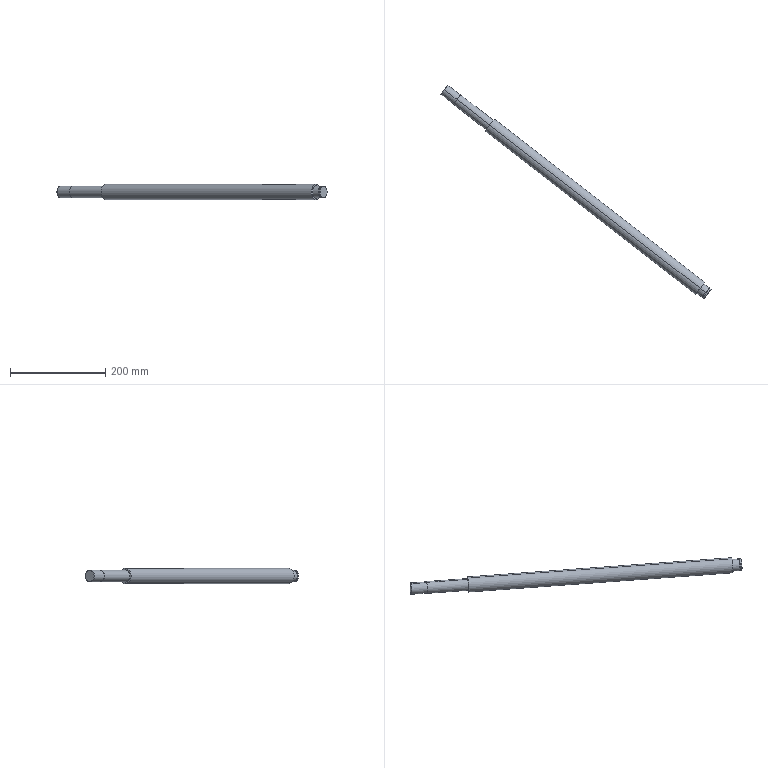Component | SolidWorks | MISUMI_BSSRK3210-800-F34-P20-1_SHAFT_MISUMI_BSSRK3210-800-F34-P20-1 | 1 solid | 27 faces | box 567.36 x 447.98 x 32 mm | volume 517409 mm3 | cylinder 12 | plane 7 | cone 4 | torus 4 | commonest cylinder face diameters 25 x6 24 x2 23.9 x2 32 x2
build123d program:
from build123d import *

# Parameters (mm, degrees)
FILLET1_R     = 0.3
FILLET2_R     = 0.5
CHAMFER1_SIZE = 0.5


with BuildPart() as part:
    # Sketch1 → Revolve1 (revolve)
    with BuildSketch(Plane.XY, mode=Mode.PRIVATE) as revolve1_sk:
        Polygon((0, 0), (700, 0), (700, 12), (666, 12), (666, 12.5), (579, 12.5), (579, 16), (20, 16), (20, 12.5), (5, 12.5), (5, 11.95), (3.65, 11.95), (3.65, 12.5), (0, 12.5), align=None)
    revolve(revolve1_sk.sketch.rotate(Axis((0, 0, 0), (1, 0, 0)), 90), axis=Axis((0, 0, 0), (1, 0, 0)))

    # Fillet1
    fillet1_edges = [part.edges().sort_by_distance(p)[0] for p in [
        (579, 0, -12.5),
    ]]
    fillet(fillet1_edges, radius=FILLET1_R)

    # Fillet2
    fillet2_edges = [part.edges().sort_by_distance(p)[0] for p in [
        (20, 0, -12.5),
    ]]
    fillet(fillet2_edges, radius=FILLET2_R)

    # Chamfer1
    chamfer1_edges = [part.edges().sort_by_distance(p)[0] for p in [
        (700, 0, -12),
        (0, 0, -12.5),
    ]]
    chamfer(chamfer1_edges, length=CHAMFER1_SIZE)


solid = part.part

# Placed as in the assembly
solid = solid.moved(Location((382.255, 447.91, 276.411), (0.7035, -0.5461, 142.183)))
STEP:
#1=COLOUR_RGB('',0.7922,0.8196,0.9333);
#2=FILL_AREA_STYLE_COLOUR('',#1);
#3=FILL_AREA_STYLE('',(#2));
#4=SURFACE_STYLE_FILL_AREA(#3);
#5=SURFACE_SIDE_STYLE('',(#4));
#6=SURFACE_STYLE_USAGE(.BOTH.,#5);
#7=PRESENTATION_STYLE_ASSIGNMENT((#6));
#8=CARTESIAN_POINT('',(15.049,17.634,11.355));
#9=VERTEX_POINT('',#8);
#10=CARTESIAN_POINT('',(15.049,17.634,10.41));
#11=VERTEX_POINT('',#10);
#12=CARTESIAN_POINT('',(15.049,17.634,10.882));
#13=DIRECTION('',(0.7899,-0.6132,-0.));
#14=DIRECTION('',(0.,0.,-1.));
#15=AXIS2_PLACEMENT_3D('',#12,#13,#14);
#16=CIRCLE('',#15,0.4724);
#17=EDGE_CURVE('',#9,#11,#16,.T.);
#18=ORIENTED_EDGE('',*,*,#17,.F.);
#19=CARTESIAN_POINT('',(15.034,17.646,11.374));
#20=VERTEX_POINT('',#19);
#21=CARTESIAN_POINT('',(15.049,17.634,11.355));
#22=DIRECTION('',(-0.5586,0.4336,0.7071));
#23=VECTOR('',#22,39.37);
#24=LINE('',#21,#23);
#25=EDGE_CURVE('',#9,#20,#24,.T.);
#26=ORIENTED_EDGE('',*,*,#25,.T.);
#27=CARTESIAN_POINT('',(15.034,17.646,10.39));
#28=VERTEX_POINT('',#27);
#29=CARTESIAN_POINT('',(15.034,17.646,10.882));
#30=DIRECTION('',(-0.7899,0.6132,0.));
#31=DIRECTION('',(0.,0.,-1.));
#32=AXIS2_PLACEMENT_3D('',#29,#30,#31);
#33=CIRCLE('',#32,0.4921);
#34=EDGE_CURVE('',#28,#20,#33,.T.);
#35=ORIENTED_EDGE('',*,*,#34,.F.);
#36=CARTESIAN_POINT('',(15.049,17.634,10.41));
#37=DIRECTION('',(-0.5586,0.4336,-0.7071));
#38=VECTOR('',#37,39.37);
#39=LINE('',#36,#38);
#40=EDGE_CURVE('',#11,#28,#39,.T.);
#41=ORIENTED_EDGE('',*,*,#40,.F.);
#42=EDGE_LOOP('',(#18,#26,#35,#41));
#43=FACE_OUTER_BOUND('',#42,.T.);
#44=CARTESIAN_POINT('',(15.049,17.634,10.882));
#45=DIRECTION('',(-0.7899,0.6132,0.));
#46=DIRECTION('',(0.,0.,-1.));
#47=AXIS2_PLACEMENT_3D('',#44,#45,#46);
#48=CONICAL_SURFACE('',#47,0.4724,0.7854);
#49=ADVANCED_FACE('',(#43),#48,.T.);
#50=CARTESIAN_POINT('',(-6.72,34.533,10.43));
#51=VERTEX_POINT('',#50);
#52=CARTESIAN_POINT('',(-6.72,34.533,11.335));
#53=VERTEX_POINT('',#52);
#54=CARTESIAN_POINT('',(-6.72,34.533,10.882));
#55=DIRECTION('',(-0.7899,0.6132,0.));
#56=DIRECTION('',(-0.,-0.,1.));
#57=AXIS2_PLACEMENT_3D('',#54,#55,#56);
#58=CIRCLE('',#57,0.4528);
#59=EDGE_CURVE('',#51,#53,#58,.T.);
#60=ORIENTED_EDGE('',*,*,#59,.F.);
#61=CARTESIAN_POINT('',(-6.705,34.521,10.41));
#62=VERTEX_POINT('',#61);
#63=CARTESIAN_POINT('',(-6.705,34.521,10.41));
#64=DIRECTION('',(0.5586,-0.4336,-0.7071));
#65=VECTOR('',#64,39.37);
#66=LINE('',#63,#65);
#67=EDGE_CURVE('',#51,#62,#66,.T.);
#68=ORIENTED_EDGE('',*,*,#67,.T.);
#69=CARTESIAN_POINT('',(-6.705,34.521,11.355));
#70=VERTEX_POINT('',#69);
#71=CARTESIAN_POINT('',(-6.705,34.521,10.882));
#72=DIRECTION('',(0.7899,-0.6132,-0.));
#73=DIRECTION('',(-0.,-0.,1.));
#74=AXIS2_PLACEMENT_3D('',#71,#72,#73);
#75=CIRCLE('',#74,0.4724);
#76=EDGE_CURVE('',#70,#62,#75,.T.);
#77=ORIENTED_EDGE('',*,*,#76,.F.);
#78=CARTESIAN_POINT('',(-6.705,34.521,11.355));
#79=DIRECTION('',(0.5586,-0.4336,0.7071));
#80=VECTOR('',#79,39.37);
#81=LINE('',#78,#80);
#82=EDGE_CURVE('',#53,#70,#81,.T.);
#83=ORIENTED_EDGE('',*,*,#82,.F.);
#84=EDGE_LOOP('',(#60,#68,#77,#83));
#85=FACE_OUTER_BOUND('',#84,.T.);
#86=CARTESIAN_POINT('',(-6.705,34.521,10.882));
#87=DIRECTION('',(0.7899,-0.6132,-0.));
#88=DIRECTION('',(-0.,-0.,1.));
#89=AXIS2_PLACEMENT_3D('',#86,#87,#88);
#90=CONICAL_SURFACE('',#89,0.4724,0.7854);
#91=ADVANCED_FACE('',(#85),#90,.T.);
#92=CARTESIAN_POINT('',(14.427,18.117,11.394));
#93=VERTEX_POINT('',#92);
#94=CARTESIAN_POINT('',(14.427,18.117,10.371));
#95=VERTEX_POINT('',#94);
#96=CARTESIAN_POINT('',(14.427,18.117,10.882));
#97=DIRECTION('',(-0.7899,0.6132,0.));
#98=DIRECTION('',(0.,0.,-1.));
#99=AXIS2_PLACEMENT_3D('',#96,#97,#98);
#100=CIRCLE('',#99,0.5118);
#101=EDGE_CURVE('',#93,#95,#100,.T.);
#102=ORIENTED_EDGE('',*,*,#101,.F.);
#103=CARTESIAN_POINT('',(14.443,18.105,11.374));
#104=VERTEX_POINT('',#103);
#105=CARTESIAN_POINT('',(14.443,18.105,11.394));
#106=DIRECTION('',(-0.6132,-0.7899,-0.));
#107=DIRECTION('',(0.7899,-0.6132,0.));
#108=AXIS2_PLACEMENT_3D('',#105,#106,#107);
#109=CIRCLE('',#108,0.01969);
#110=EDGE_CURVE('',#93,#104,#109,.T.);
#111=ORIENTED_EDGE('',*,*,#110,.T.);
#112=CARTESIAN_POINT('',(14.443,18.105,10.39));
#113=VERTEX_POINT('',#112);
#114=CARTESIAN_POINT('',(14.443,18.105,10.882));
#115=DIRECTION('',(0.7899,-0.6132,-0.));
#116=DIRECTION('',(0.,0.,-1.));
#117=AXIS2_PLACEMENT_3D('',#114,#115,#116);
#118=CIRCLE('',#117,0.4921);
#119=EDGE_CURVE('',#113,#104,#118,.T.);
#120=ORIENTED_EDGE('',*,*,#119,.F.);
#121=CARTESIAN_POINT('',(14.443,18.105,10.371));
#122=DIRECTION('',(0.6132,0.7899,0.));
#123=DIRECTION('',(-0.7899,0.6132,0.));
#124=AXIS2_PLACEMENT_3D('',#121,#122,#123);
#125=CIRCLE('',#124,0.01969);
#126=EDGE_CURVE('',#95,#113,#125,.T.);
#127=ORIENTED_EDGE('',*,*,#126,.F.);
#128=EDGE_LOOP('',(#102,#111,#120,#127));
#129=FACE_OUTER_BOUND('',#128,.T.);
#130=CARTESIAN_POINT('',(14.443,18.105,10.882));
#131=DIRECTION('',(-0.7899,0.6132,0.));
#132=DIRECTION('',(0.,0.,-1.));
#133=AXIS2_PLACEMENT_3D('',#130,#131,#132);
#134=TOROIDAL_SURFACE('',#133,0.5118,0.01969);
#135=ADVANCED_FACE('',(#129),#134,.F.);
#136=CARTESIAN_POINT('',(-2.957,31.612,10.378));
#137=VERTEX_POINT('',#136);
#138=CARTESIAN_POINT('',(-2.957,31.612,11.386));
#139=VERTEX_POINT('',#138);
#140=CARTESIAN_POINT('',(-2.957,31.612,10.882));
#141=DIRECTION('',(0.7899,-0.6132,-0.));
#142=DIRECTION('',(-0.,-0.,1.));
#143=AXIS2_PLACEMENT_3D('',#140,#141,#142);
#144=CIRCLE('',#143,0.5039);
#145=EDGE_CURVE('',#137,#139,#144,.T.);
#146=ORIENTED_EDGE('',*,*,#145,.F.);
#147=CARTESIAN_POINT('',(-2.967,31.619,10.39));
#148=VERTEX_POINT('',#147);
#149=CARTESIAN_POINT('',(-2.967,31.619,10.378));
#150=DIRECTION('',(-0.6132,-0.7899,-0.));
#151=DIRECTION('',(0.7899,-0.6132,0.));
#152=AXIS2_PLACEMENT_3D('',#149,#150,#151);
#153=CIRCLE('',#152,0.01181);
#154=EDGE_CURVE('',#137,#148,#153,.T.);
#155=ORIENTED_EDGE('',*,*,#154,.T.);
#156=CARTESIAN_POINT('',(-2.967,31.619,11.374));
#157=VERTEX_POINT('',#156);
#158=CARTESIAN_POINT('',(-2.967,31.619,10.882));
#159=DIRECTION('',(-0.7899,0.6132,0.));
#160=DIRECTION('',(-0.,-0.,1.));
#161=AXIS2_PLACEMENT_3D('',#158,#159,#160);
#162=CIRCLE('',#161,0.4921);
#163=EDGE_CURVE('',#157,#148,#162,.T.);
#164=ORIENTED_EDGE('',*,*,#163,.F.);
#165=CARTESIAN_POINT('',(-2.967,31.619,11.386));
#166=DIRECTION('',(0.6132,0.7899,0.));
#167=DIRECTION('',(-0.7899,0.6132,0.));
#168=AXIS2_PLACEMENT_3D('',#165,#166,#167);
#169=CIRCLE('',#168,0.01181);
#170=EDGE_CURVE('',#139,#157,#169,.T.);
#171=ORIENTED_EDGE('',*,*,#170,.F.);
#172=EDGE_LOOP('',(#146,#155,#164,#171));
#173=FACE_OUTER_BOUND('',#172,.T.);
#174=CARTESIAN_POINT('',(-2.967,31.619,10.882));
#175=DIRECTION('',(0.7899,-0.6132,-0.));
#176=DIRECTION('',(-0.,-0.,1.));
#177=AXIS2_PLACEMENT_3D('',#174,#175,#176);
#178=TOROIDAL_SURFACE('',#177,0.5039,0.01181);
#179=ADVANCED_FACE('',(#173),#178,.F.);
#180=CARTESIAN_POINT('',(-5.663,33.713,11.374));
#181=VERTEX_POINT('',#180);
#182=CARTESIAN_POINT('',(-5.663,33.713,10.39));
#183=VERTEX_POINT('',#182);
#184=CARTESIAN_POINT('',(-5.663,33.713,10.882));
#185=DIRECTION('',(0.7899,-0.6132,-0.));
#186=DIRECTION('',(-0.,-0.,1.));
#187=AXIS2_PLACEMENT_3D('',#184,#185,#186);
#188=CIRCLE('',#187,0.4921);
#189=EDGE_CURVE('',#181,#183,#188,.T.);
#190=ORIENTED_EDGE('',*,*,#189,.T.);
#191=CARTESIAN_POINT('',(15.049,17.634,10.39));
#192=DIRECTION('',(0.7899,-0.6132,-0.));
#193=VECTOR('',#192,39.37);
#194=LINE('',#191,#193);
#195=EDGE_CURVE('',#183,#148,#194,.T.);
#196=ORIENTED_EDGE('',*,*,#195,.T.);
#197=CARTESIAN_POINT('',(-2.967,31.619,10.882));
#198=DIRECTION('',(-0.7899,0.6132,0.));
#199=DIRECTION('',(-0.,-0.,1.));
#200=AXIS2_PLACEMENT_3D('',#197,#198,#199);
#201=CIRCLE('',#200,0.4921);
#202=EDGE_CURVE('',#148,#157,#201,.T.);
#203=ORIENTED_EDGE('',*,*,#202,.T.);
#204=CARTESIAN_POINT('',(15.049,17.634,11.374));
#205=DIRECTION('',(0.7899,-0.6132,-0.));
#206=VECTOR('',#205,39.37);
#207=LINE('',#204,#206);
#208=EDGE_CURVE('',#181,#157,#207,.T.);
#209=ORIENTED_EDGE('',*,*,#208,.F.);
#210=EDGE_LOOP('',(#190,#196,#203,#209));
#211=FACE_OUTER_BOUND('',#210,.T.);
#212=CARTESIAN_POINT('',(15.049,17.634,10.882));
#213=DIRECTION('',(0.7899,-0.6132,-0.));
#214=DIRECTION('',(-0.,-0.,1.));
#215=AXIS2_PLACEMENT_3D('',#212,#213,#214);
#216=CYLINDRICAL_SURFACE('',#215,0.4921);
#217=ADVANCED_FACE('',(#211),#216,.T.);
#218=ORIENTED_EDGE('',*,*,#76,.T.);
#219=CARTESIAN_POINT('',(-5.663,33.713,10.41));
#220=VERTEX_POINT('',#219);
#221=CARTESIAN_POINT('',(15.049,17.634,10.41));
#222=DIRECTION('',(0.7899,-0.6132,-0.));
#223=VECTOR('',#222,39.37);
#224=LINE('',#221,#223);
#225=EDGE_CURVE('',#62,#220,#224,.T.);
#226=ORIENTED_EDGE('',*,*,#225,.T.);
#227=CARTESIAN_POINT('',(-5.663,33.713,11.355));
#228=VERTEX_POINT('',#227);
#229=CARTESIAN_POINT('',(-5.663,33.713,10.882));
#230=DIRECTION('',(0.7899,-0.6132,-0.));
#231=DIRECTION('',(-0.,-0.,1.));
#232=AXIS2_PLACEMENT_3D('',#229,#230,#231);
#233=CIRCLE('',#232,0.4724);
#234=EDGE_CURVE('',#228,#220,#233,.T.);
#235=ORIENTED_EDGE('',*,*,#234,.F.);
#236=CARTESIAN_POINT('',(15.049,17.634,11.355));
#237=DIRECTION('',(0.7899,-0.6132,-0.));
#238=VECTOR('',#237,39.37);
#239=LINE('',#236,#238);
#240=EDGE_CURVE('',#70,#228,#239,.T.);
#241=ORIENTED_EDGE('',*,*,#240,.F.);
#242=EDGE_LOOP('',(#218,#226,#235,#241));
#243=FACE_OUTER_BOUND('',#242,.T.);
#244=CARTESIAN_POINT('',(15.049,17.634,10.882));
#245=DIRECTION('',(0.7899,-0.6132,-0.));
#246=DIRECTION('',(-0.,-0.,1.));
#247=AXIS2_PLACEMENT_3D('',#244,#245,#246);
#248=CYLINDRICAL_SURFACE('',#247,0.4724);
#249=ADVANCED_FACE('',(#243),#248,.T.);
#250=CARTESIAN_POINT('',(14.936,17.722,11.374));
#251=VERTEX_POINT('',#250);
#252=CARTESIAN_POINT('',(14.936,17.722,10.39));
#253=VERTEX_POINT('',#252);
#254=CARTESIAN_POINT('',(14.936,17.722,10.882));
#255=DIRECTION('',(0.7899,-0.6132,-0.));
#256=DIRECTION('',(-0.,-0.,1.));
#257=AXIS2_PLACEMENT_3D('',#254,#255,#256);
#258=CIRCLE('',#257,0.4921);
#259=EDGE_CURVE('',#251,#253,#258,.T.);
#260=ORIENTED_EDGE('',*,*,#259,.T.);
#261=CARTESIAN_POINT('',(15.049,17.634,10.39));
#262=DIRECTION('',(0.7899,-0.6132,-0.));
#263=VECTOR('',#262,39.37);
#264=LINE('',#261,#263);
#265=EDGE_CURVE('',#253,#28,#264,.T.);
#266=ORIENTED_EDGE('',*,*,#265,.T.);
#267=ORIENTED_EDGE('',*,*,#34,.T.);
#268=CARTESIAN_POINT('',(15.049,17.634,11.374));
#269=DIRECTION('',(0.7899,-0.6132,-0.));
#270=VECTOR('',#269,39.37);
#271=LINE('',#268,#270);
#272=EDGE_CURVE('',#251,#20,#271,.T.);
#273=ORIENTED_EDGE('',*,*,#272,.F.);
#274=EDGE_LOOP('',(#260,#266,#267,#273));
#275=FACE_OUTER_BOUND('',#274,.T.);
#276=CARTESIAN_POINT('',(15.049,17.634,10.882));
#277=DIRECTION('',(0.7899,-0.6132,-0.));
#278=DIRECTION('',(-0.,-0.,1.));
#279=AXIS2_PLACEMENT_3D('',#276,#277,#278);
#280=CYLINDRICAL_SURFACE('',#279,0.4921);
#281=ADVANCED_FACE('',(#275),#280,.T.);
#282=CARTESIAN_POINT('',(14.894,17.755,11.353));
#283=VERTEX_POINT('',#282);
#284=CARTESIAN_POINT('',(14.894,17.755,10.412));
#285=VERTEX_POINT('',#284);
#286=CARTESIAN_POINT('',(14.894,17.755,10.882));
#287=DIRECTION('',(0.7899,-0.6132,-0.));
#288=DIRECTION('',(-0.,-0.,1.));
#289=AXIS2_PLACEMENT_3D('',#286,#287,#288);
#290=CIRCLE('',#289,0.4705);
#291=EDGE_CURVE('',#283,#285,#290,.T.);
#292=ORIENTED_EDGE('',*,*,#291,.T.);
#293=CARTESIAN_POINT('',(14.936,17.722,10.412));
#294=VERTEX_POINT('',#293);
#295=CARTESIAN_POINT('',(15.049,17.634,10.412));
#296=DIRECTION('',(0.7899,-0.6132,-0.));
#297=VECTOR('',#296,39.37);
#298=LINE('',#295,#297);
#299=EDGE_CURVE('',#285,#294,#298,.T.);
#300=ORIENTED_EDGE('',*,*,#299,.T.);
#301=CARTESIAN_POINT('',(14.936,17.722,11.353));
#302=VERTEX_POINT('',#301);
#303=CARTESIAN_POINT('',(14.936,17.722,10.882));
#304=DIRECTION('',(0.7899,-0.6132,-0.));
#305=DIRECTION('',(-0.,-0.,1.));
#306=AXIS2_PLACEMENT_3D('',#303,#304,#305);
#307=CIRCLE('',#306,0.4705);
#308=EDGE_CURVE('',#302,#294,#307,.T.);
#309=ORIENTED_EDGE('',*,*,#308,.F.);
#310=CARTESIAN_POINT('',(15.049,17.634,11.353));
#311=DIRECTION('',(0.7899,-0.6132,-0.));
#312=VECTOR('',#311,39.37);
#313=LINE('',#310,#312);
#314=EDGE_CURVE('',#283,#302,#313,.T.);
#315=ORIENTED_EDGE('',*,*,#314,.F.);
#316=EDGE_LOOP('',(#292,#300,#309,#315));
#317=FACE_OUTER_BOUND('',#316,.T.);
#318=CARTESIAN_POINT('',(15.049,17.634,10.882));
#319=DIRECTION('',(0.7899,-0.6132,-0.));
#320=DIRECTION('',(-0.,-0.,1.));
#321=AXIS2_PLACEMENT_3D('',#318,#319,#320);
#322=CYLINDRICAL_SURFACE('',#321,0.4705);
#323=ADVANCED_FACE('',(#317),#322,.T.);
#324=CARTESIAN_POINT('',(14.443,18.105,10.882));
#325=DIRECTION('',(0.7899,-0.6132,-0.));
#326=DIRECTION('',(0.,0.,-1.));
#327=AXIS2_PLACEMENT_3D('',#324,#325,#326);
#328=CIRCLE('',#327,0.4921);
#329=EDGE_CURVE('',#104,#113,#328,.T.);
#330=ORIENTED_EDGE('',*,*,#329,.T.);
#331=CARTESIAN_POINT('',(14.894,17.755,10.39));
#332=VERTEX_POINT('',#331);
#333=CARTESIAN_POINT('',(15.049,17.634,10.39));
#334=DIRECTION('',(0.7899,-0.6132,-0.));
#335=VECTOR('',#334,39.37);
#336=LINE('',#333,#335);
#337=EDGE_CURVE('',#113,#332,#336,.T.);
#338=ORIENTED_EDGE('',*,*,#337,.T.);
#339=CARTESIAN_POINT('',(14.894,17.755,11.374));
#340=VERTEX_POINT('',#339);
#341=CARTESIAN_POINT('',(14.894,17.755,10.882));
#342=DIRECTION('',(0.7899,-0.6132,-0.));
#343=DIRECTION('',(-0.,-0.,1.));
#344=AXIS2_PLACEMENT_3D('',#341,#342,#343);
#345=CIRCLE('',#344,0.4921);
#346=EDGE_CURVE('',#340,#332,#345,.T.);
#347=ORIENTED_EDGE('',*,*,#346,.F.);
#348=CARTESIAN_POINT('',(15.049,17.634,11.374));
#349=DIRECTION('',(0.7899,-0.6132,-0.));
#350=VECTOR('',#349,39.37);
#351=LINE('',#348,#350);
#352=EDGE_CURVE('',#104,#340,#351,.T.);
#353=ORIENTED_EDGE('',*,*,#352,.F.);
#354=EDGE_LOOP('',(#330,#338,#347,#353));
#355=FACE_OUTER_BOUND('',#354,.T.);
#356=CARTESIAN_POINT('',(15.049,17.634,10.882));
#357=DIRECTION('',(0.7899,-0.6132,-0.));
#358=DIRECTION('',(-0.,-0.,1.));
#359=AXIS2_PLACEMENT_3D('',#356,#357,#358);
#360=CYLINDRICAL_SURFACE('',#359,0.4921);
#361=ADVANCED_FACE('',(#355),#360,.T.);
#362=CARTESIAN_POINT('',(-2.957,31.612,11.512));
#363=VERTEX_POINT('',#362);
#364=CARTESIAN_POINT('',(-2.957,31.612,10.252));
#365=VERTEX_POINT('',#364);
#366=CARTESIAN_POINT('',(-2.957,31.612,10.882));
#367=DIRECTION('',(0.7899,-0.6132,-0.));
#368=DIRECTION('',(-0.,-0.,1.));
#369=AXIS2_PLACEMENT_3D('',#366,#367,#368);
#370=CIRCLE('',#369,0.6299);
#371=EDGE_CURVE('',#363,#365,#370,.T.);
#372=ORIENTED_EDGE('',*,*,#371,.T.);
#373=CARTESIAN_POINT('',(14.427,18.117,10.252));
#374=VERTEX_POINT('',#373);
#375=CARTESIAN_POINT('',(15.049,17.634,10.252));
#376=DIRECTION('',(0.7899,-0.6132,-0.));
#377=VECTOR('',#376,39.37);
#378=LINE('',#375,#377);
#379=EDGE_CURVE('',#365,#374,#378,.T.);
#380=ORIENTED_EDGE('',*,*,#379,.T.);
#381=CARTESIAN_POINT('',(14.427,18.117,11.512));
#382=VERTEX_POINT('',#381);
#383=CARTESIAN_POINT('',(14.427,18.117,10.882));
#384=DIRECTION('',(0.7899,-0.6132,-0.));
#385=DIRECTION('',(-0.,-0.,1.));
#386=AXIS2_PLACEMENT_3D('',#383,#384,#385);
#387=CIRCLE('',#386,0.6299);
#388=EDGE_CURVE('',#382,#374,#387,.T.);
#389=ORIENTED_EDGE('',*,*,#388,.F.);
#390=CARTESIAN_POINT('',(15.049,17.634,11.512));
#391=DIRECTION('',(0.7899,-0.6132,-0.));
#392=VECTOR('',#391,39.37);
#393=LINE('',#390,#392);
#394=EDGE_CURVE('',#363,#382,#393,.T.);
#395=ORIENTED_EDGE('',*,*,#394,.F.);
#396=EDGE_LOOP('',(#372,#380,#389,#395));
#397=FACE_OUTER_BOUND('',#396,.T.);
#398=CARTESIAN_POINT('',(15.049,17.634,10.882));
#399=DIRECTION('',(0.7899,-0.6132,-0.));
#400=DIRECTION('',(-0.,-0.,1.));
#401=AXIS2_PLACEMENT_3D('',#398,#399,#400);
#402=CYLINDRICAL_SURFACE('',#401,0.6299);
#403=ADVANCED_FACE('',(#397),#402,.T.);
#404=CARTESIAN_POINT('',(-2.957,31.612,10.882));
#405=DIRECTION('',(0.7899,-0.6132,-0.));
#406=DIRECTION('',(-0.,-0.,1.));
#407=AXIS2_PLACEMENT_3D('',#404,#405,#406);
#408=CIRCLE('',#407,0.5039);
#409=EDGE_CURVE('',#139,#137,#408,.T.);
#410=ORIENTED_EDGE('',*,*,#409,.T.);
#411=ORIENTED_EDGE('',*,*,#145,.T.);
#412=EDGE_LOOP('',(#410,#411));
#413=FACE_BOUND('',#412,.T.);
#414=ORIENTED_EDGE('',*,*,#371,.F.);
#415=CARTESIAN_POINT('',(-2.957,31.612,10.882));
#416=DIRECTION('',(0.7899,-0.6132,-0.));
#417=DIRECTION('',(-0.,-0.,1.));
#418=AXIS2_PLACEMENT_3D('',#415,#416,#417);
#419=CIRCLE('',#418,0.6299);
#420=EDGE_CURVE('',#365,#363,#419,.T.);
#421=ORIENTED_EDGE('',*,*,#420,.F.);
#422=EDGE_LOOP('',(#414,#421));
#423=FACE_OUTER_BOUND('',#422,.T.);
#424=CARTESIAN_POINT('',(-3.259,31.223,10.882));
#425=DIRECTION('',(0.7899,-0.6132,-0.));
#426=DIRECTION('',(-0.,-0.,1.));
#427=AXIS2_PLACEMENT_3D('',#424,#425,#426);
#428=PLANE('',#427);
#429=ADVANCED_FACE('',(#413,#423),#428,.F.);
#430=ORIENTED_EDGE('',*,*,#379,.F.);
#431=ORIENTED_EDGE('',*,*,#420,.T.);
#432=ORIENTED_EDGE('',*,*,#394,.T.);
#433=CARTESIAN_POINT('',(14.427,18.117,10.882));
#434=DIRECTION('',(0.7899,-0.6132,-0.));
#435=DIRECTION('',(-0.,-0.,1.));
#436=AXIS2_PLACEMENT_3D('',#433,#434,#435);
#437=CIRCLE('',#436,0.6299);
#438=EDGE_CURVE('',#374,#382,#437,.T.);
#439=ORIENTED_EDGE('',*,*,#438,.F.);
#440=EDGE_LOOP('',(#430,#431,#432,#439));
#441=FACE_OUTER_BOUND('',#440,.T.);
#442=CARTESIAN_POINT('',(15.049,17.634,10.882));
#443=DIRECTION('',(0.7899,-0.6132,-0.));
#444=DIRECTION('',(-0.,-0.,1.));
#445=AXIS2_PLACEMENT_3D('',#442,#443,#444);
#446=CYLINDRICAL_SURFACE('',#445,0.6299);
#447=ADVANCED_FACE('',(#441),#446,.T.);
#448=CARTESIAN_POINT('',(14.427,18.117,10.882));
#449=DIRECTION('',(-0.7899,0.6132,0.));
#450=DIRECTION('',(0.,0.,-1.));
#451=AXIS2_PLACEMENT_3D('',#448,#449,#450);
#452=CIRCLE('',#451,0.5118);
#453=EDGE_CURVE('',#95,#93,#452,.T.);
#454=ORIENTED_EDGE('',*,*,#453,.T.);
#455=ORIENTED_EDGE('',*,*,#101,.T.);
#456=EDGE_LOOP('',(#454,#455));
#457=FACE_BOUND('',#456,.T.);
#458=ORIENTED_EDGE('',*,*,#388,.T.);
#459=ORIENTED_EDGE('',*,*,#438,.T.);
#460=EDGE_LOOP('',(#458,#459));
#461=FACE_OUTER_BOUND('',#460,.T.);
#462=CARTESIAN_POINT('',(14.041,17.619,10.882));
#463=DIRECTION('',(-0.7899,0.6132,0.));
#464=DIRECTION('',(0.,0.,-1.));
#465=AXIS2_PLACEMENT_3D('',#462,#463,#464);
#466=PLANE('',#465);
#467=ADVANCED_FACE('',(#457,#461),#466,.F.);
#468=ORIENTED_EDGE('',*,*,#337,.F.);
#469=ORIENTED_EDGE('',*,*,#119,.T.);
#470=ORIENTED_EDGE('',*,*,#352,.T.);
#471=CARTESIAN_POINT('',(14.894,17.755,10.882));
#472=DIRECTION('',(0.7899,-0.6132,-0.));
#473=DIRECTION('',(-0.,-0.,1.));
#474=AXIS2_PLACEMENT_3D('',#471,#472,#473);
#475=CIRCLE('',#474,0.4921);
#476=EDGE_CURVE('',#332,#340,#475,.T.);
#477=ORIENTED_EDGE('',*,*,#476,.F.);
#478=EDGE_LOOP('',(#468,#469,#470,#477));
#479=FACE_OUTER_BOUND('',#478,.T.);
#480=CARTESIAN_POINT('',(15.049,17.634,10.882));
#481=DIRECTION('',(0.7899,-0.6132,-0.));
#482=DIRECTION('',(-0.,-0.,1.));
#483=AXIS2_PLACEMENT_3D('',#480,#481,#482);
#484=CYLINDRICAL_SURFACE('',#483,0.4921);
#485=ADVANCED_FACE('',(#479),#484,.T.);
#486=ORIENTED_EDGE('',*,*,#291,.F.);
#487=CARTESIAN_POINT('',(14.894,17.755,10.882));
#488=DIRECTION('',(0.7899,-0.6132,-0.));
#489=DIRECTION('',(-0.,-0.,1.));
#490=AXIS2_PLACEMENT_3D('',#487,#488,#489);
#491=CIRCLE('',#490,0.4705);
#492=EDGE_CURVE('',#285,#283,#491,.T.);
#493=ORIENTED_EDGE('',*,*,#492,.F.);
#494=EDGE_LOOP('',(#486,#493));
#495=FACE_BOUND('',#494,.T.);
#496=ORIENTED_EDGE('',*,*,#346,.T.);
#497=ORIENTED_EDGE('',*,*,#476,.T.);
#498=EDGE_LOOP('',(#496,#497));
#499=FACE_OUTER_BOUND('',#498,.T.);
#500=CARTESIAN_POINT('',(14.592,17.366,10.882));
#501=DIRECTION('',(-0.7899,0.6132,0.));
#502=DIRECTION('',(0.,0.,-1.));
#503=AXIS2_PLACEMENT_3D('',#500,#501,#502);
#504=PLANE('',#503);
#505=ADVANCED_FACE('',(#495,#499),#504,.F.);
#506=ORIENTED_EDGE('',*,*,#299,.F.);
#507=ORIENTED_EDGE('',*,*,#492,.T.);
#508=ORIENTED_EDGE('',*,*,#314,.T.);
#509=CARTESIAN_POINT('',(14.936,17.722,10.882));
#510=DIRECTION('',(0.7899,-0.6132,-0.));
#511=DIRECTION('',(-0.,-0.,1.));
#512=AXIS2_PLACEMENT_3D('',#509,#510,#511);
#513=CIRCLE('',#512,0.4705);
#514=EDGE_CURVE('',#294,#302,#513,.T.);
#515=ORIENTED_EDGE('',*,*,#514,.F.);
#516=EDGE_LOOP('',(#506,#507,#508,#515));
#517=FACE_OUTER_BOUND('',#516,.T.);
#518=CARTESIAN_POINT('',(15.049,17.634,10.882));
#519=DIRECTION('',(0.7899,-0.6132,-0.));
#520=DIRECTION('',(-0.,-0.,1.));
#521=AXIS2_PLACEMENT_3D('',#518,#519,#520);
#522=CYLINDRICAL_SURFACE('',#521,0.4705);
#523=ADVANCED_FACE('',(#517),#522,.T.);
#524=ORIENTED_EDGE('',*,*,#259,.F.);
#525=CARTESIAN_POINT('',(14.936,17.722,10.882));
#526=DIRECTION('',(0.7899,-0.6132,-0.));
#527=DIRECTION('',(-0.,-0.,1.));
#528=AXIS2_PLACEMENT_3D('',#525,#526,#527);
#529=CIRCLE('',#528,0.4921);
#530=EDGE_CURVE('',#253,#251,#529,.T.);
#531=ORIENTED_EDGE('',*,*,#530,.F.);
#532=EDGE_LOOP('',(#524,#531));
#533=FACE_OUTER_BOUND('',#532,.T.);
#534=ORIENTED_EDGE('',*,*,#308,.T.);
#535=ORIENTED_EDGE('',*,*,#514,.T.);
#536=EDGE_LOOP('',(#534,#535));
#537=FACE_BOUND('',#536,.T.);
#538=CARTESIAN_POINT('',(14.647,17.351,10.882));
#539=DIRECTION('',(0.7899,-0.6132,-0.));
#540=DIRECTION('',(-0.,-0.,1.));
#541=AXIS2_PLACEMENT_3D('',#538,#539,#540);
#542=PLANE('',#541);
#543=ADVANCED_FACE('',(#533,#537),#542,.F.);
#544=ORIENTED_EDGE('',*,*,#265,.F.);
#545=ORIENTED_EDGE('',*,*,#530,.T.);
#546=ORIENTED_EDGE('',*,*,#272,.T.);
#547=CARTESIAN_POINT('',(15.034,17.646,10.882));
#548=DIRECTION('',(-0.7899,0.6132,0.));
#549=DIRECTION('',(0.,0.,-1.));
#550=AXIS2_PLACEMENT_3D('',#547,#548,#549);
#551=CIRCLE('',#550,0.4921);
#552=EDGE_CURVE('',#20,#28,#551,.T.);
#553=ORIENTED_EDGE('',*,*,#552,.T.);
#554=EDGE_LOOP('',(#544,#545,#546,#553));
#555=FACE_OUTER_BOUND('',#554,.T.);
#556=CARTESIAN_POINT('',(15.049,17.634,10.882));
#557=DIRECTION('',(0.7899,-0.6132,-0.));
#558=DIRECTION('',(-0.,-0.,1.));
#559=AXIS2_PLACEMENT_3D('',#556,#557,#558);
#560=CYLINDRICAL_SURFACE('',#559,0.4921);
#561=ADVANCED_FACE('',(#555),#560,.T.);
#562=CARTESIAN_POINT('',(15.049,17.634,10.882));
#563=DIRECTION('',(0.7899,-0.6132,-0.));
#564=DIRECTION('',(0.,0.,-1.));
#565=AXIS2_PLACEMENT_3D('',#562,#563,#564);
#566=CIRCLE('',#565,0.4724);
#567=EDGE_CURVE('',#11,#9,#566,.T.);
#568=ORIENTED_EDGE('',*,*,#567,.T.);
#569=ORIENTED_EDGE('',*,*,#17,.T.);
#570=EDGE_LOOP('',(#568,#569));
#571=FACE_OUTER_BOUND('',#570,.T.);
#572=CARTESIAN_POINT('',(14.748,17.246,10.882));
#573=DIRECTION('',(-0.7899,0.6132,0.));
#574=DIRECTION('',(0.,0.,-1.));
#575=AXIS2_PLACEMENT_3D('',#572,#573,#574);
#576=PLANE('',#575);
#577=ADVANCED_FACE('',(#571),#576,.F.);
#578=CARTESIAN_POINT('',(-6.72,34.533,10.882));
#579=DIRECTION('',(-0.7899,0.6132,0.));
#580=DIRECTION('',(-0.,-0.,1.));
#581=AXIS2_PLACEMENT_3D('',#578,#579,#580);
#582=CIRCLE('',#581,0.4528);
#583=EDGE_CURVE('',#53,#51,#582,.T.);
#584=ORIENTED_EDGE('',*,*,#583,.T.);
#585=ORIENTED_EDGE('',*,*,#59,.T.);
#586=EDGE_LOOP('',(#584,#585));
#587=FACE_OUTER_BOUND('',#586,.T.);
#588=CARTESIAN_POINT('',(-6.72,34.533,10.882));
#589=DIRECTION('',(0.7899,-0.6132,-0.));
#590=DIRECTION('',(-0.,-0.,1.));
#591=AXIS2_PLACEMENT_3D('',#588,#589,#590);
#592=PLANE('',#591);
#593=ADVANCED_FACE('',(#587),#592,.F.);
#594=ORIENTED_EDGE('',*,*,#225,.F.);
#595=CARTESIAN_POINT('',(-6.705,34.521,10.882));
#596=DIRECTION('',(0.7899,-0.6132,-0.));
#597=DIRECTION('',(-0.,-0.,1.));
#598=AXIS2_PLACEMENT_3D('',#595,#596,#597);
#599=CIRCLE('',#598,0.4724);
#600=EDGE_CURVE('',#62,#70,#599,.T.);
#601=ORIENTED_EDGE('',*,*,#600,.T.);
#602=ORIENTED_EDGE('',*,*,#240,.T.);
#603=CARTESIAN_POINT('',(-5.663,33.713,10.882));
#604=DIRECTION('',(0.7899,-0.6132,-0.));
#605=DIRECTION('',(-0.,-0.,1.));
#606=AXIS2_PLACEMENT_3D('',#603,#604,#605);
#607=CIRCLE('',#606,0.4724);
#608=EDGE_CURVE('',#220,#228,#607,.T.);
#609=ORIENTED_EDGE('',*,*,#608,.F.);
#610=EDGE_LOOP('',(#594,#601,#602,#609));
#611=FACE_OUTER_BOUND('',#610,.T.);
#612=CARTESIAN_POINT('',(15.049,17.634,10.882));
#613=DIRECTION('',(0.7899,-0.6132,-0.));
#614=DIRECTION('',(-0.,-0.,1.));
#615=AXIS2_PLACEMENT_3D('',#612,#613,#614);
#616=CYLINDRICAL_SURFACE('',#615,0.4724);
#617=ADVANCED_FACE('',(#611),#616,.T.);
#618=ORIENTED_EDGE('',*,*,#189,.F.);
#619=CARTESIAN_POINT('',(-5.663,33.713,10.882));
#620=DIRECTION('',(0.7899,-0.6132,-0.));
#621=DIRECTION('',(-0.,-0.,1.));
#622=AXIS2_PLACEMENT_3D('',#619,#620,#621);
#623=CIRCLE('',#622,0.4921);
#624=EDGE_CURVE('',#183,#181,#623,.T.);
#625=ORIENTED_EDGE('',*,*,#624,.F.);
#626=EDGE_LOOP('',(#618,#625));
#627=FACE_OUTER_BOUND('',#626,.T.);
#628=ORIENTED_EDGE('',*,*,#234,.T.);
#629=ORIENTED_EDGE('',*,*,#608,.T.);
#630=EDGE_LOOP('',(#628,#629));
#631=FACE_BOUND('',#630,.T.);
#632=CARTESIAN_POINT('',(-5.953,33.339,10.882));
#633=DIRECTION('',(0.7899,-0.6132,-0.));
#634=DIRECTION('',(-0.,-0.,1.));
#635=AXIS2_PLACEMENT_3D('',#632,#633,#634);
#636=PLANE('',#635);
#637=ADVANCED_FACE('',(#627,#631),#636,.F.);
#638=ORIENTED_EDGE('',*,*,#195,.F.);
#639=ORIENTED_EDGE('',*,*,#624,.T.);
#640=ORIENTED_EDGE('',*,*,#208,.T.);
#641=ORIENTED_EDGE('',*,*,#163,.T.);
#642=EDGE_LOOP('',(#638,#639,#640,#641));
#643=FACE_OUTER_BOUND('',#642,.T.);
#644=CARTESIAN_POINT('',(15.049,17.634,10.882));
#645=DIRECTION('',(0.7899,-0.6132,-0.));
#646=DIRECTION('',(-0.,-0.,1.));
#647=AXIS2_PLACEMENT_3D('',#644,#645,#646);
#648=CYLINDRICAL_SURFACE('',#647,0.4921);
#649=ADVANCED_FACE('',(#643),#648,.T.);
#650=ORIENTED_EDGE('',*,*,#154,.F.);
#651=ORIENTED_EDGE('',*,*,#409,.F.);
#652=ORIENTED_EDGE('',*,*,#170,.T.);
#653=ORIENTED_EDGE('',*,*,#202,.F.);
#654=EDGE_LOOP('',(#650,#651,#652,#653));
#655=FACE_OUTER_BOUND('',#654,.T.);
#656=CARTESIAN_POINT('',(-2.967,31.619,10.882));
#657=DIRECTION('',(0.7899,-0.6132,-0.));
#658=DIRECTION('',(-0.,-0.,1.));
#659=AXIS2_PLACEMENT_3D('',#656,#657,#658);
#660=TOROIDAL_SURFACE('',#659,0.5039,0.01181);
#661=ADVANCED_FACE('',(#655),#660,.F.);
#662=ORIENTED_EDGE('',*,*,#110,.F.);
#663=ORIENTED_EDGE('',*,*,#453,.F.);
#664=ORIENTED_EDGE('',*,*,#126,.T.);
#665=ORIENTED_EDGE('',*,*,#329,.F.);
#666=EDGE_LOOP('',(#662,#663,#664,#665));
#667=FACE_OUTER_BOUND('',#666,.T.);
#668=CARTESIAN_POINT('',(14.443,18.105,10.882));
#669=DIRECTION('',(-0.7899,0.6132,0.));
#670=DIRECTION('',(0.,0.,-1.));
#671=AXIS2_PLACEMENT_3D('',#668,#669,#670);
#672=TOROIDAL_SURFACE('',#671,0.5118,0.01969);
#673=ADVANCED_FACE('',(#667),#672,.F.);
#674=ORIENTED_EDGE('',*,*,#67,.F.);
#675=ORIENTED_EDGE('',*,*,#583,.F.);
#676=ORIENTED_EDGE('',*,*,#82,.T.);
#677=ORIENTED_EDGE('',*,*,#600,.F.);
#678=EDGE_LOOP('',(#674,#675,#676,#677));
#679=FACE_OUTER_BOUND('',#678,.T.);
#680=CARTESIAN_POINT('',(-6.705,34.521,10.882));
#681=DIRECTION('',(0.7899,-0.6132,-0.));
#682=DIRECTION('',(-0.,-0.,1.));
#683=AXIS2_PLACEMENT_3D('',#680,#681,#682);
#684=CONICAL_SURFACE('',#683,0.4724,0.7854);
#685=ADVANCED_FACE('',(#679),#684,.T.);
#686=ORIENTED_EDGE('',*,*,#25,.F.);
#687=ORIENTED_EDGE('',*,*,#567,.F.);
#688=ORIENTED_EDGE('',*,*,#40,.T.);
#689=ORIENTED_EDGE('',*,*,#552,.F.);
#690=EDGE_LOOP('',(#686,#687,#688,#689));
#691=FACE_OUTER_BOUND('',#690,.T.);
#692=CARTESIAN_POINT('',(15.049,17.634,10.882));
#693=DIRECTION('',(-0.7899,0.6132,0.));
#694=DIRECTION('',(0.,0.,-1.));
#695=AXIS2_PLACEMENT_3D('',#692,#693,#694);
#696=CONICAL_SURFACE('',#695,0.4724,0.7854);
#697=ADVANCED_FACE('',(#691),#696,.T.);
#698=CLOSED_SHELL('',(#49,#91,#135,#179,#217,#249,#281,#323,#361,#403,#429,#447,#467,#485,#505,#523,#543,#561,#577,#593,#617,#637,#649,#661,#673,#685,#697));
#699=MANIFOLD_SOLID_BREP('',#698);
#700=STYLED_ITEM('',(#7),#699);
#701=(LENGTH_UNIT()NAMED_UNIT(*)SI_UNIT($,.METRE.));
#702=LENGTH_MEASURE_WITH_UNIT(LENGTH_MEASURE(0.0254),#701);
#703=DIMENSIONAL_EXPONENTS(1.,0.,0.,0.,0.,0.,0.);
#704=(CONVERSION_BASED_UNIT('',#702)LENGTH_UNIT()NAMED_UNIT(#703));
#705=UNCERTAINTY_MEASURE_WITH_UNIT(LENGTH_MEASURE(0.00001),#704,'','');
#706=(NAMED_UNIT(*)PLANE_ANGLE_UNIT()SI_UNIT($,.RADIAN.));
#707=(NAMED_UNIT(*)SI_UNIT($,.STERADIAN.)SOLID_ANGLE_UNIT());
#708=(GEOMETRIC_REPRESENTATION_CONTEXT(3)GLOBAL_UNCERTAINTY_ASSIGNED_CONTEXT((#705))GLOBAL_UNIT_ASSIGNED_CONTEXT((#704,#706,#707))REPRESENTATION_CONTEXT('',''));
#709=MECHANICAL_DESIGN_GEOMETRIC_PRESENTATION_REPRESENTATION('',(#700),#708);
#710=PRESENTATION_LAYER_ASSIGNMENT('','',(#700));
#711=CARTESIAN_POINT('',(0.,0.,0.));
#712=DIRECTION('',(0.,0.,1.));
#713=DIRECTION('',(1.,0.,0.));
#714=AXIS2_PLACEMENT_3D('',#711,#712,#713);
#715=(LENGTH_UNIT()NAMED_UNIT(*)SI_UNIT($,.METRE.));
#716=LENGTH_MEASURE_WITH_UNIT(LENGTH_MEASURE(0.0254),#715);
#717=DIMENSIONAL_EXPONENTS(1.,0.,0.,0.,0.,0.,0.);
#718=(CONVERSION_BASED_UNIT('',#716)LENGTH_UNIT()NAMED_UNIT(#717));
#719=UNCERTAINTY_MEASURE_WITH_UNIT(LENGTH_MEASURE(0.00001),#718,'','');
#720=(NAMED_UNIT(*)PLANE_ANGLE_UNIT()SI_UNIT($,.RADIAN.));
#721=(NAMED_UNIT(*)SI_UNIT($,.STERADIAN.)SOLID_ANGLE_UNIT());
#722=(GEOMETRIC_REPRESENTATION_CONTEXT(3)GLOBAL_UNCERTAINTY_ASSIGNED_CONTEXT((#719))GLOBAL_UNIT_ASSIGNED_CONTEXT((#718,#720,#721))REPRESENTATION_CONTEXT('',''));
#723=ADVANCED_BREP_SHAPE_REPRESENTATION('',(#699,#714),#722);